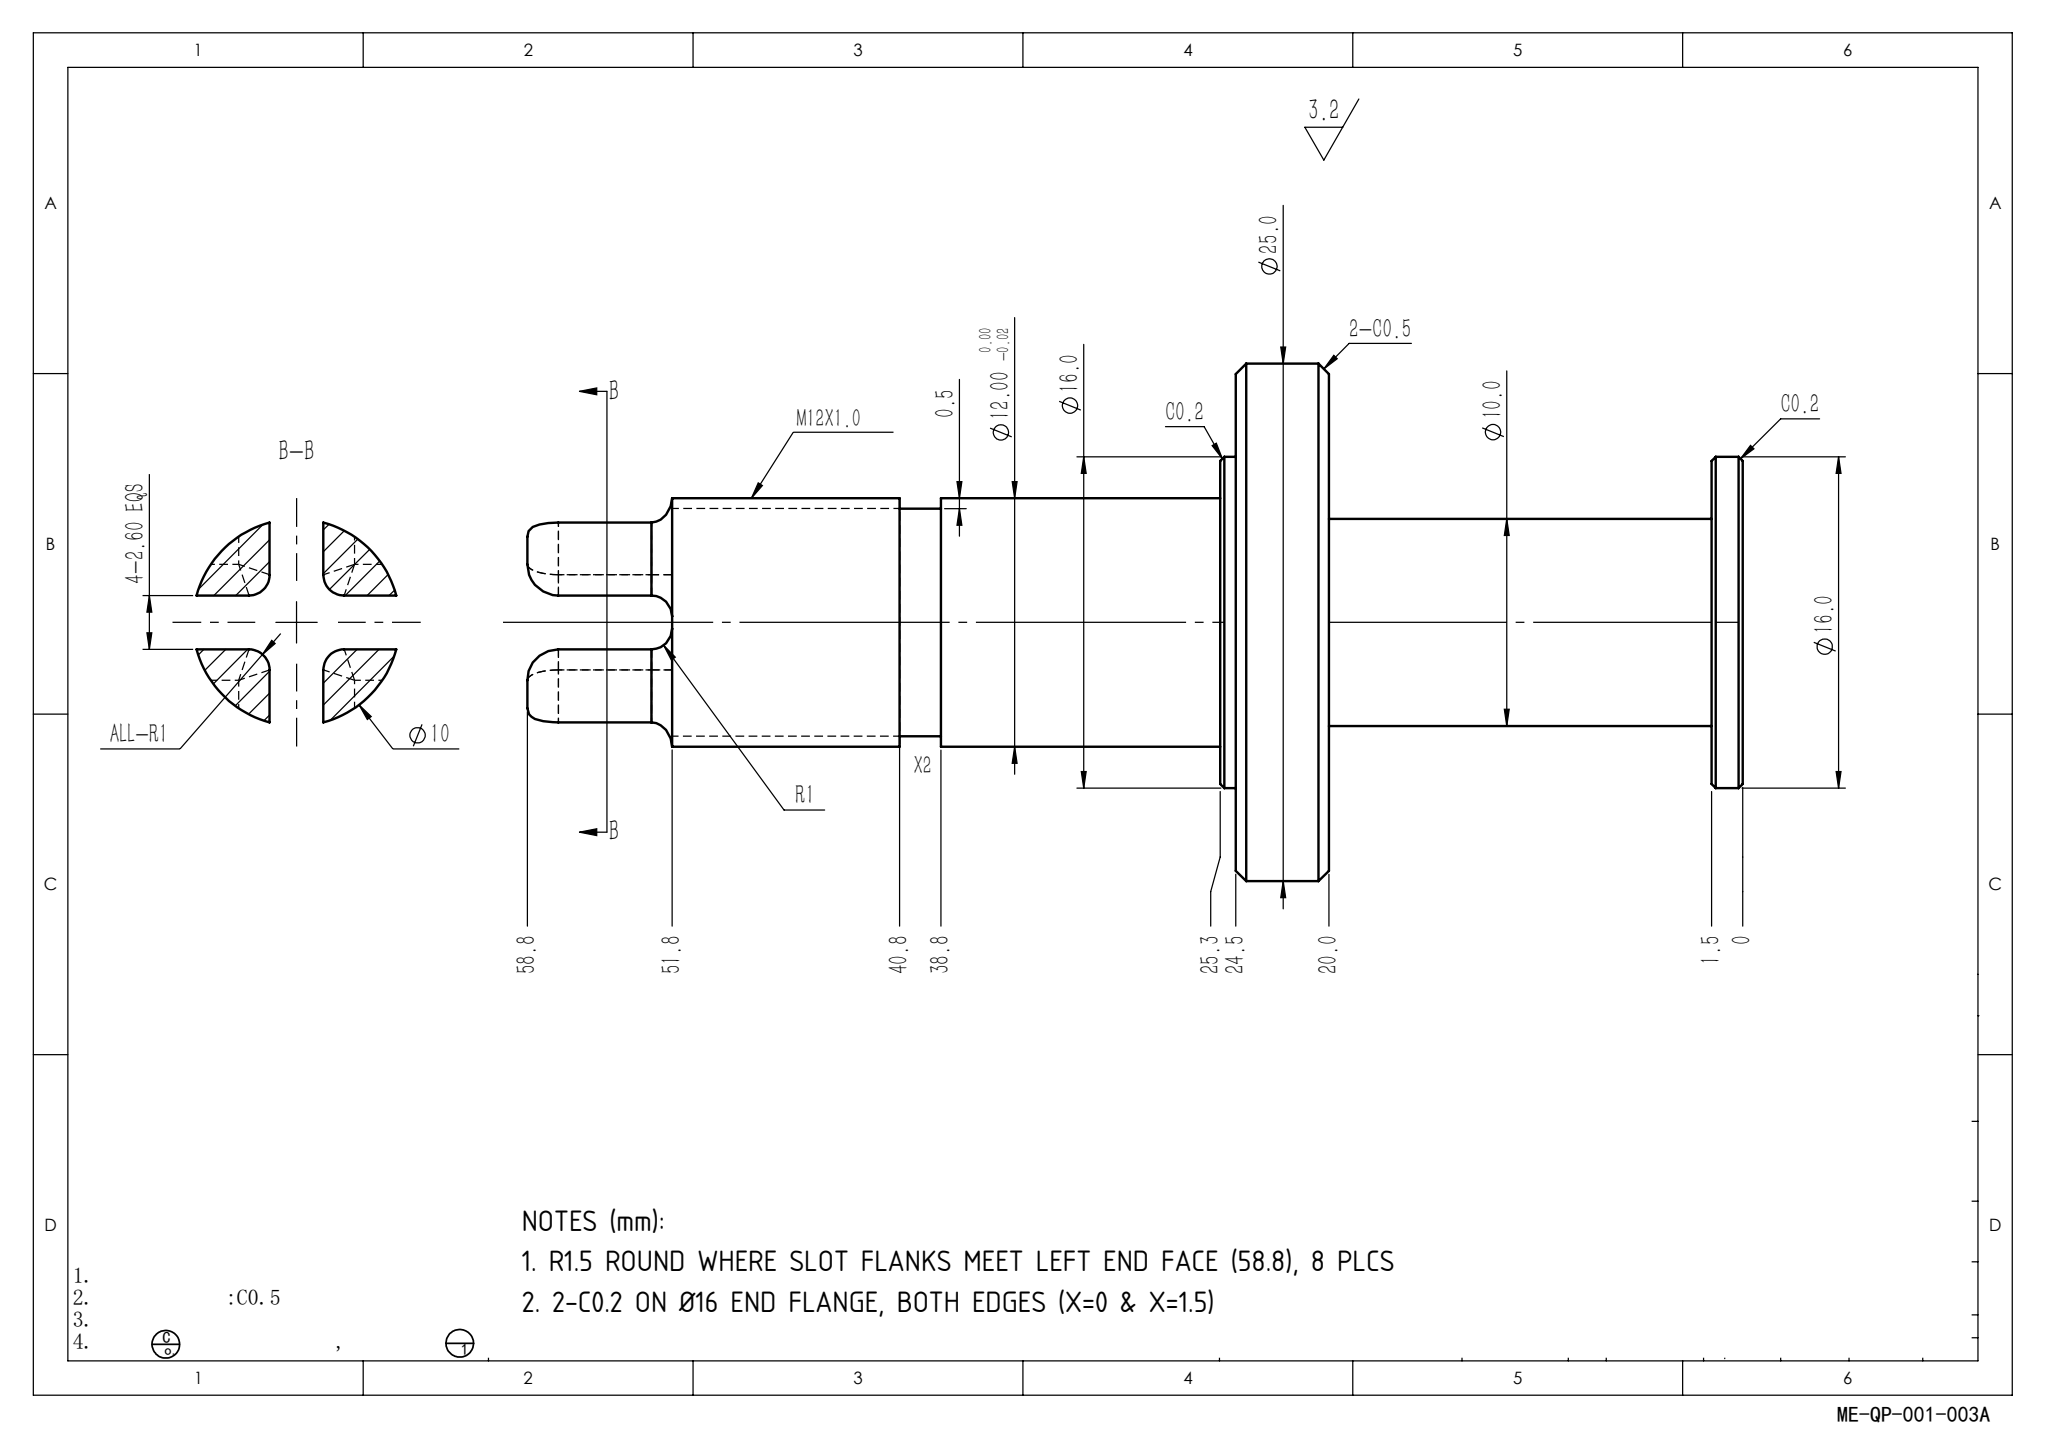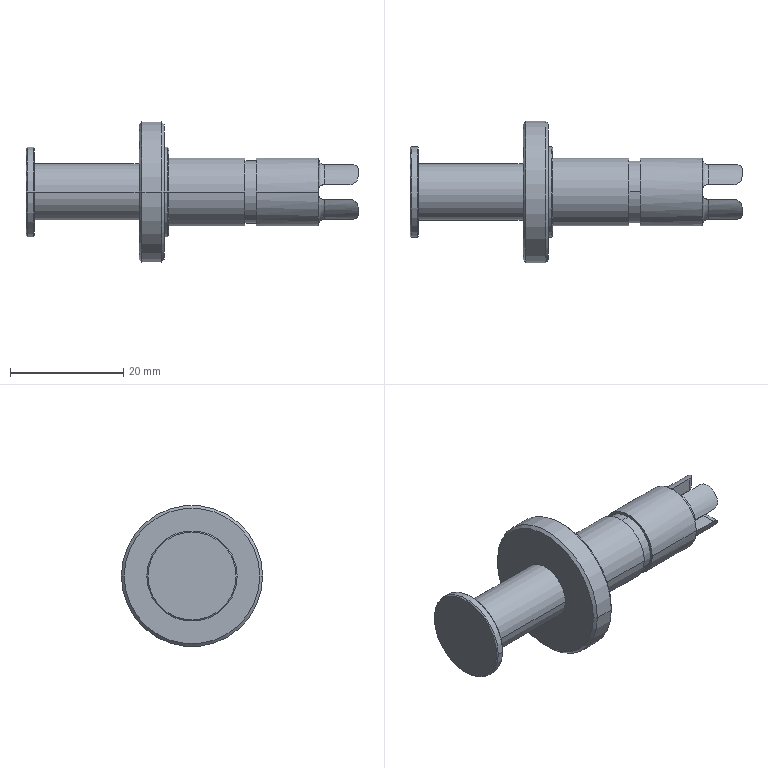Part | SolidWorks | mm | 1 solid | 80 faces | box 58.75 x 25 x 25 mm | volume 7284 mm3 | cylinder 38 | plane 20 | cone 10 | torus 8 | spline 4 | commonest cylinder face diameters 2 x12 3 x8 10 x6 16 x4 12 x4 25 x2 11 x2
Drawing notes:
R1.5 ROUND WHERE SLOT FLANKS MEET LEFT END FACE (58.8), 8 PLCS | from the solid: Ø3.0 cyl, axes y & z, x=57.25 (1.5 from end face x=58.75), at y/z=9.7 & 15.3 (slot flanks 11.2/13.8), 4 entries x2 = 8
2-C0.2 ON Ø16 END FLANGE, BOTH EDGES (X=0 & X=1.5) | from the solid: cones 90 deg incl, ref dia 16.0, count 2; Ø16 disc between planes x=0 and x=1.5